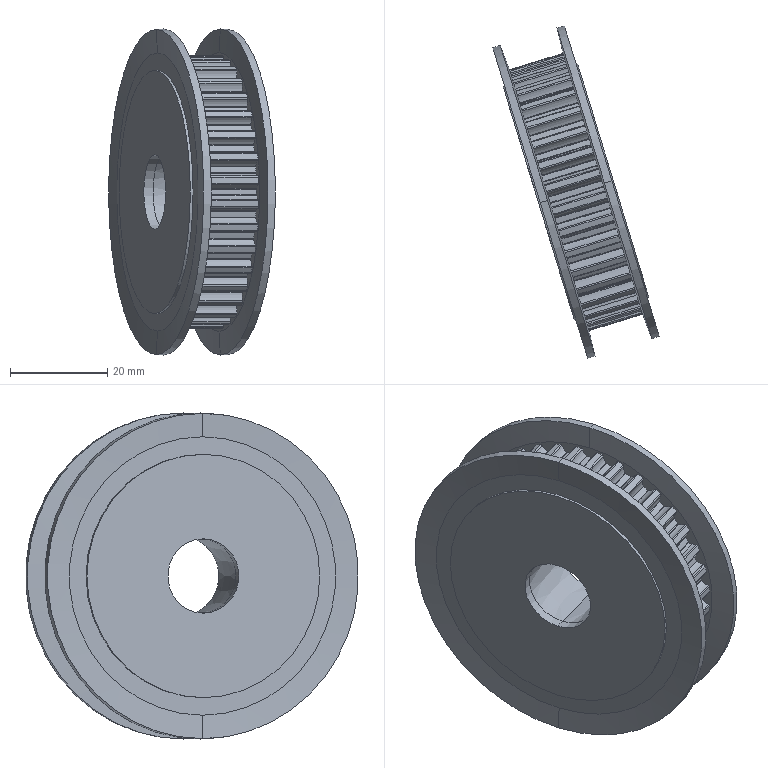Component | SolidWorks | v1ZHXTPTLA36P5M100_E_14SB1-1_v1ZHXTPTLA36P5M100_E_14_bodySB1-1 | 1 solid | 371 faces | box 34.22 x 68.39 x 67 mm | volume 36677 mm3 | cylinder 335 | cone 30 | plane 6 | commonest cylinder face diameters 0.5 x88 0.4 x82 6.64 x78 52.53 x37 56.15 x36 4.02 x8 50 x4 15.3 x2